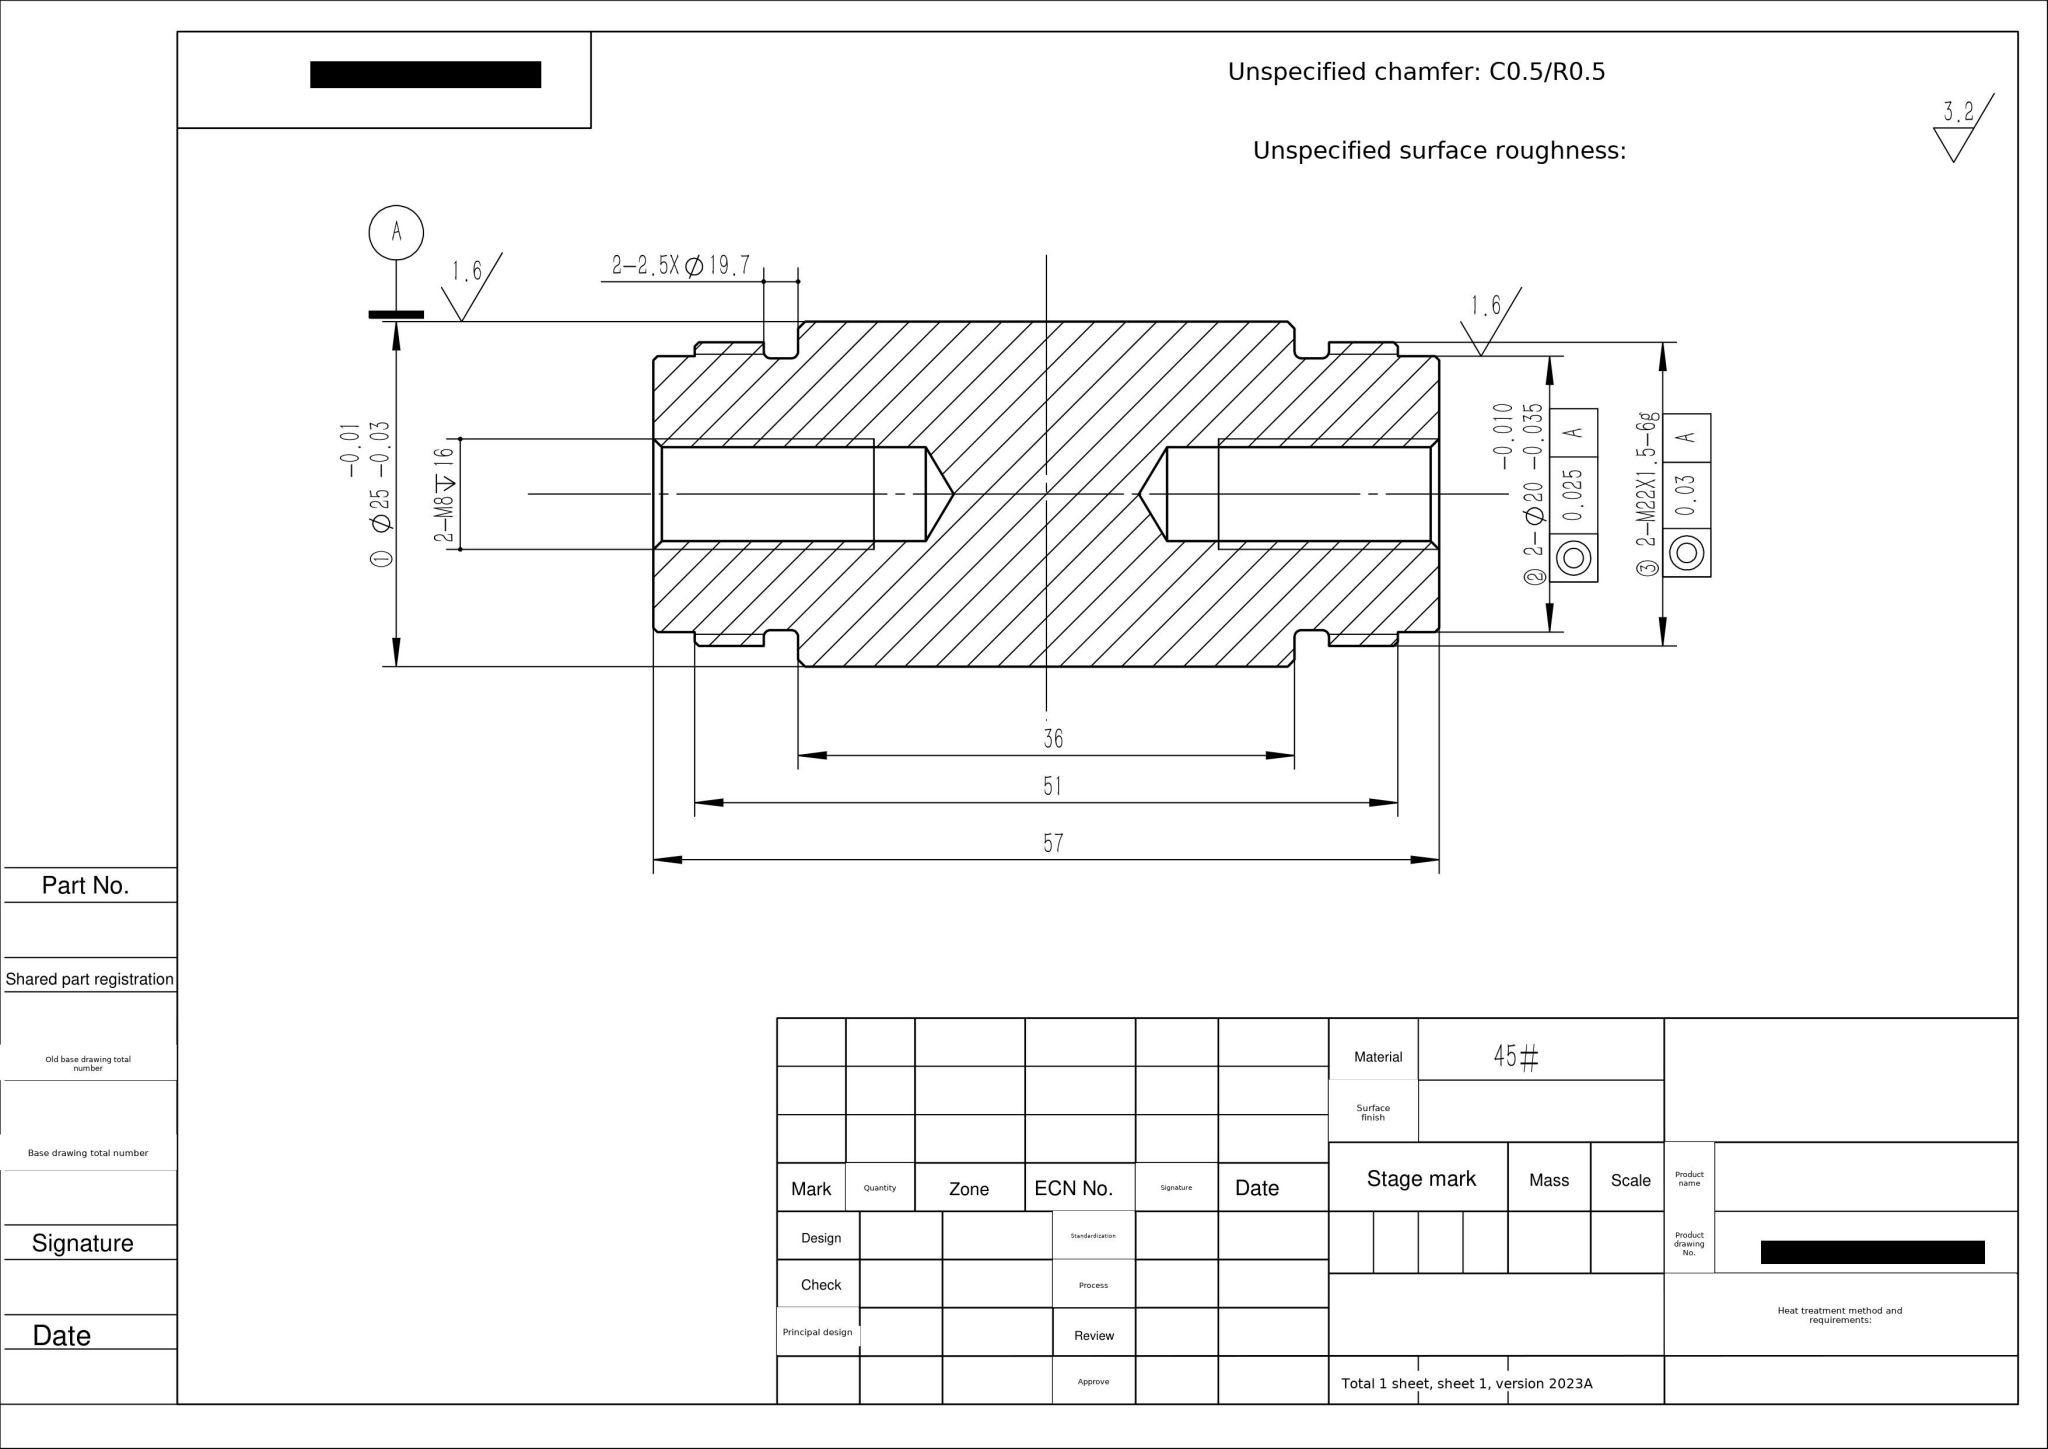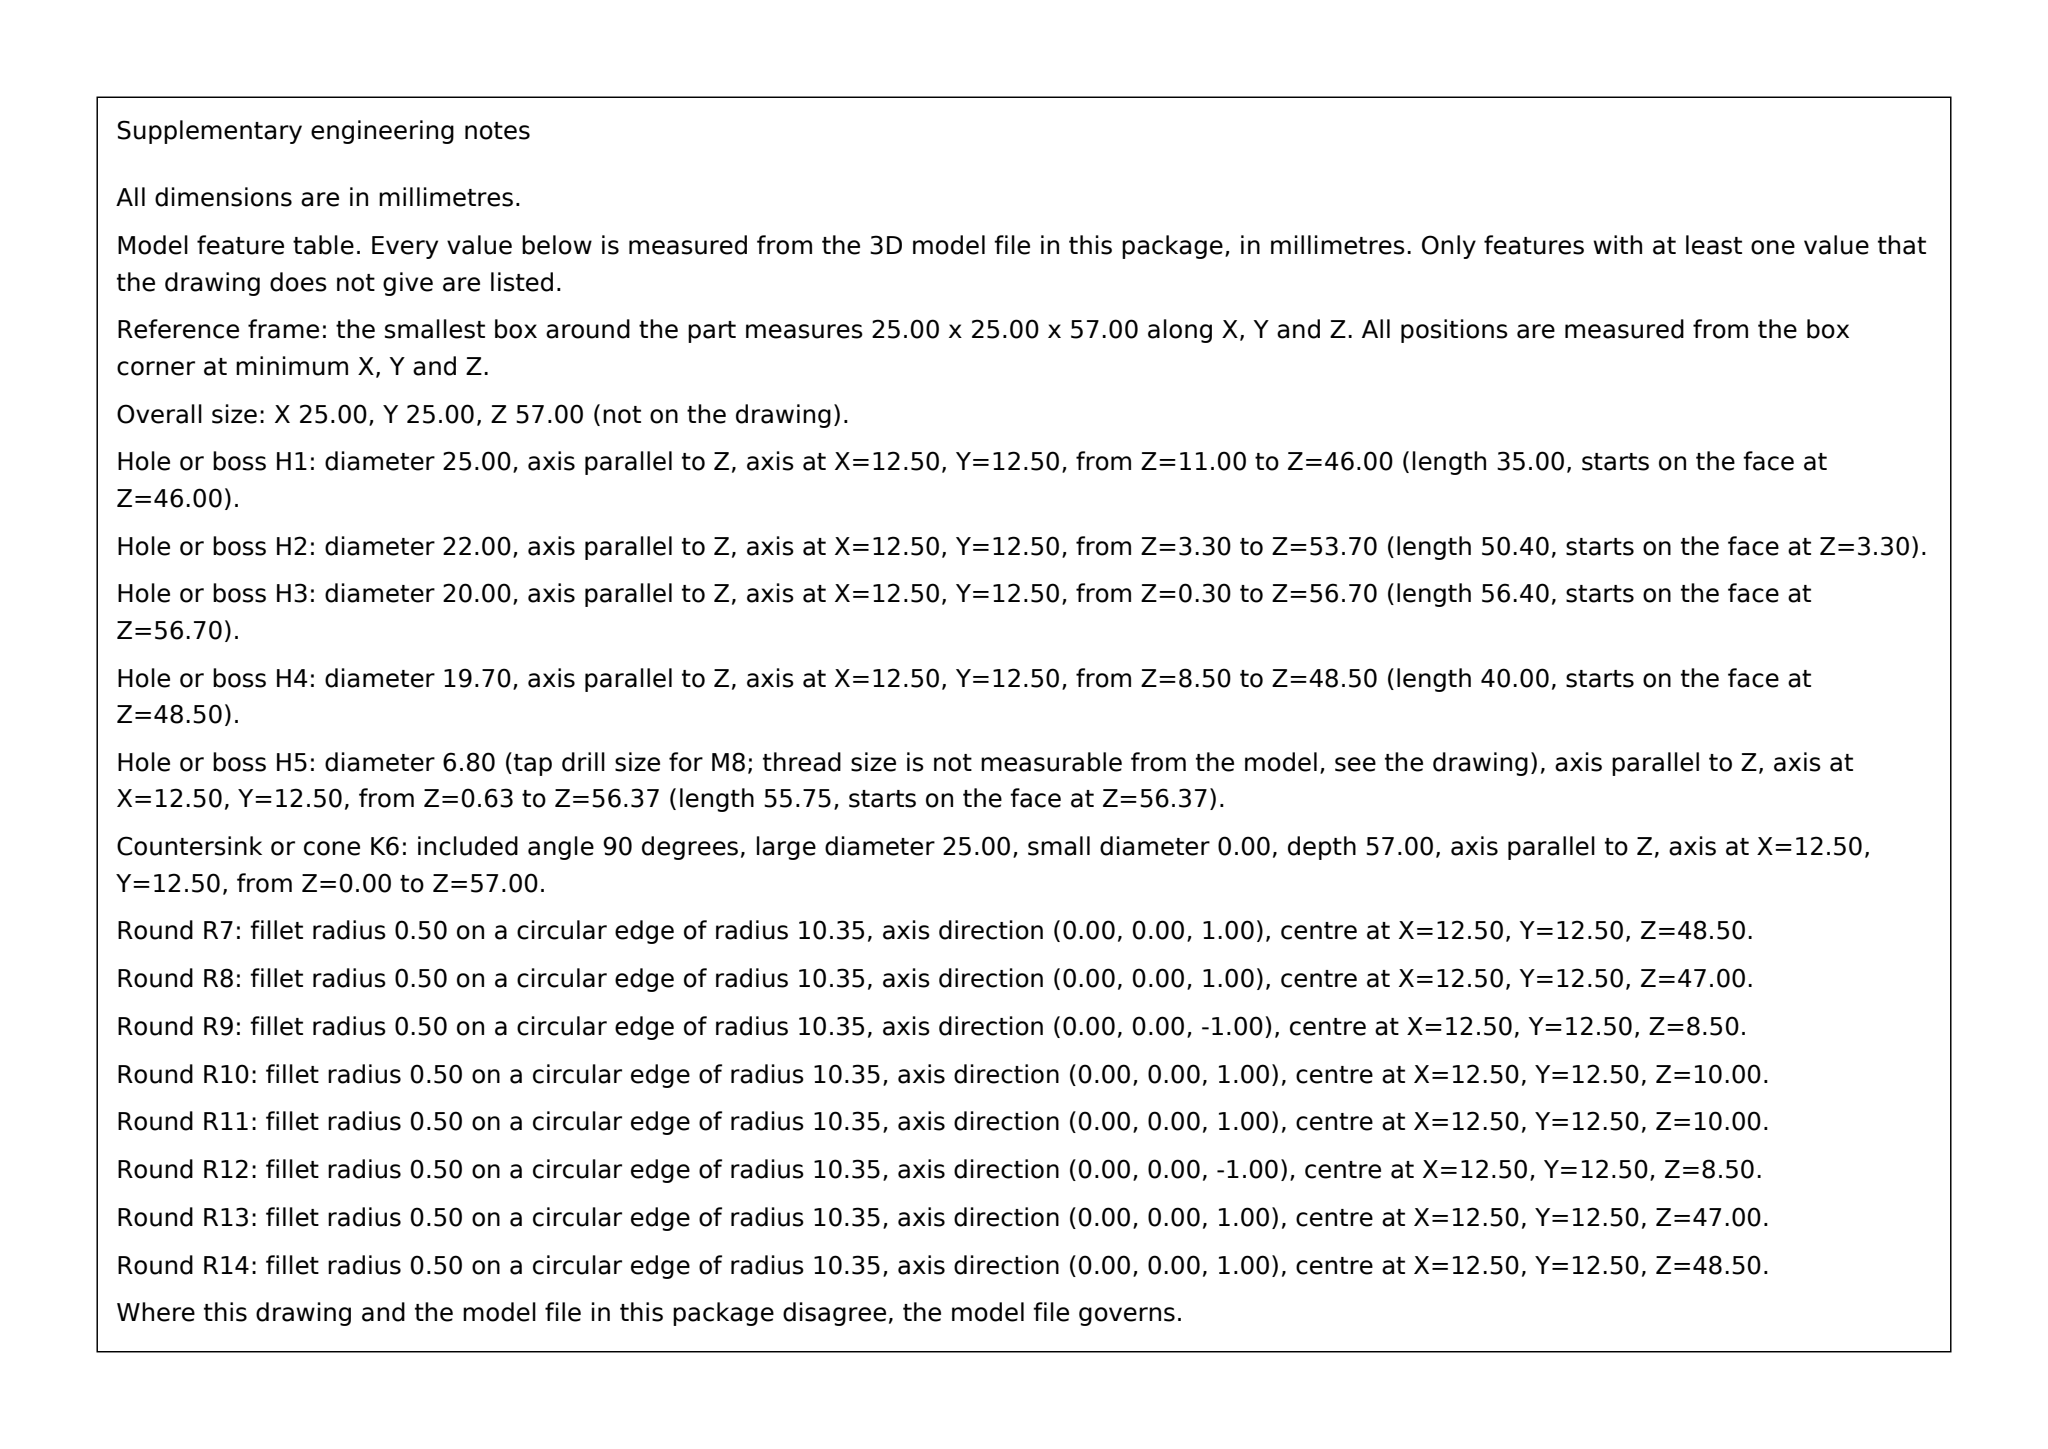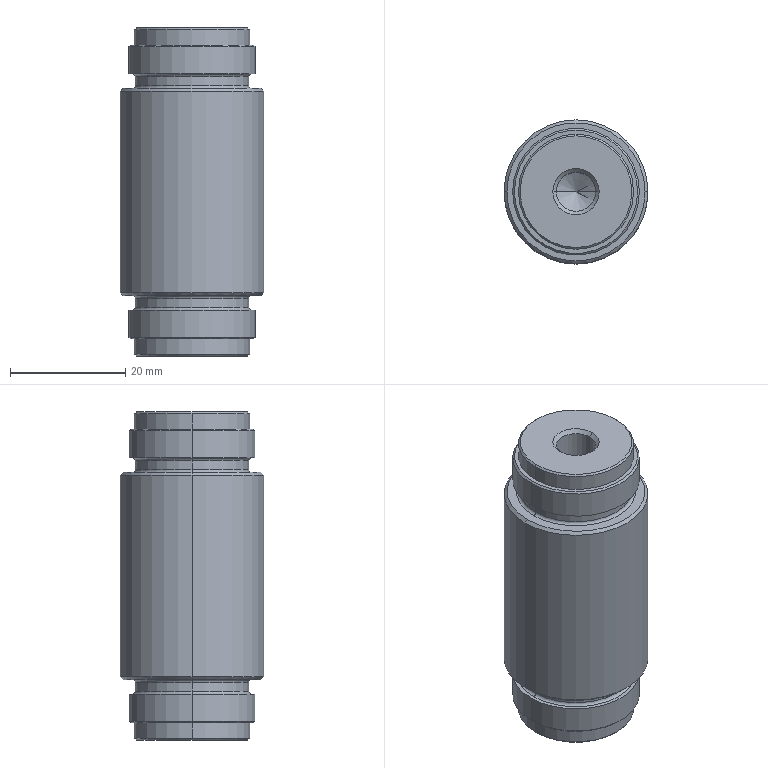Part | SolidWorks | mm | material 45# | 1 solid | 54 faces | box 25 x 25 x 57 mm | volume 23371 mm3 | cone 20 | cylinder 18 | torus 8 | plane 8 | commonest cylinder face diameters 22 x4 20 x4 6.8 x4 19.7 x4 25 x2
build123d program:
from build123d import *

# Parameters (mm, degrees)
SKETCH1_R                   = 12.5
BOSS_EXTRUDE1_DEPTH         = 18
CHAMFER1_SIZE               = 0.5
SKETCH2_R                   = 11
BOSS_EXTRUDE2_DEPTH         = 7.5
SKETCH3_R                   = 10
BOSS_EXTRUDE3_DEPTH         = 3
CHAMFER2_SIZE               = 0.3
M8_TAPPED_HOLE1_D           = 6.8
M8_TAPPED_HOLE1_DEPTH       = 19.75
M8_TAPPED_HOLE1_CSINK_D     = 8.05
M8_TAPPED_HOLE1_CSINK_ANGLE = 90
M8_TAPPED_HOLE1_TIP         = 2.043
M8_TAPPED_HOLE2_D           = 6.8
M8_TAPPED_HOLE2_DEPTH       = 19.75
M8_TAPPED_HOLE2_CSINK_D     = 8.05
M8_TAPPED_HOLE2_CSINK_ANGLE = 90
M8_TAPPED_HOLE2_TIP         = 2.043
SKETCH8_OUTSIDE_W           = 40.414
SKETCH8_OUTSIDE_H           = 40.414
SKETCH8_OUTSIDE_R           = 9.85
CUT_EXTRUDE1_DEPTH          = 2.5
FILLET1_R                   = 0.5


with BuildPart() as part:
    # Sketch1 → Boss-Extrude1 (new, symmetric)
    with BuildSketch(Plane.XY):
        Circle(SKETCH1_R)
    extrude(amount=BOSS_EXTRUDE1_DEPTH, both=True)

    # Chamfer1
    chamfer1_edges = [part.edges().sort_by_distance(p)[0] for p in [
        (-12.5, 0, -18),
        (-12.5, 0, 18),
    ]]
    chamfer(chamfer1_edges, length=CHAMFER1_SIZE)

    # Sketch2 → Boss-Extrude2 (add)
    with BuildSketch(Plane.XY.offset(18)):
        Circle(SKETCH2_R)
    boss_extrude2 = extrude(amount=BOSS_EXTRUDE2_DEPTH)

    # Mirror1: Boss-Extrude2 across plane
    add(boss_extrude2.mirror(Plane.XY))

    # Sketch3 → Boss-Extrude3 (add)
    with BuildSketch(Plane.XY.offset(25.5)):
        Circle(SKETCH3_R)
    boss_extrude3 = extrude(amount=BOSS_EXTRUDE3_DEPTH)

    # Mirror2: Boss-Extrude3 across plane
    add(boss_extrude3.mirror(Plane.XY))

    # Chamfer2
    chamfer2_edges = [part.edges().sort_by_distance(p)[0] for p in [
        (-11, 0, 25.5),
        (-11, 0, -25.5),
        (-10, 0, 28.5),
        (-10, 0, -28.5),
    ]]
    chamfer(chamfer2_edges, length=CHAMFER2_SIZE)

    # M8 Tapped Hole1
    with Locations(Plane.XY.offset(28.5)):
        with Locations((0, 0)):
            CounterSinkHole(M8_TAPPED_HOLE1_D / 2, M8_TAPPED_HOLE1_CSINK_D / 2, depth=M8_TAPPED_HOLE1_DEPTH, counter_sink_angle=M8_TAPPED_HOLE1_CSINK_ANGLE)
            with Locations((0, 0, -(M8_TAPPED_HOLE1_DEPTH + M8_TAPPED_HOLE1_TIP / 2))):  # 118° drill point
                Cone(0, M8_TAPPED_HOLE1_D / 2, M8_TAPPED_HOLE1_TIP, mode=Mode.SUBTRACT)

    # M8 Tapped Hole2
    with Locations(Plane(origin=(0, 0, -28.5), x_dir=(-1, 0, 0), z_dir=(0, 0, -1))):
        with Locations((0, 0)):
            CounterSinkHole(M8_TAPPED_HOLE2_D / 2, M8_TAPPED_HOLE2_CSINK_D / 2, depth=M8_TAPPED_HOLE2_DEPTH, counter_sink_angle=M8_TAPPED_HOLE2_CSINK_ANGLE)
            with Locations((0, 0, -(M8_TAPPED_HOLE2_DEPTH + M8_TAPPED_HOLE2_TIP / 2))):  # 118° drill point
                Cone(0, M8_TAPPED_HOLE2_D / 2, M8_TAPPED_HOLE2_TIP, mode=Mode.SUBTRACT)

    # Sketch8 outside → Cut-Extrude1 (cut)
    with BuildSketch(Plane.XY.offset(18)):
        Rectangle(SKETCH8_OUTSIDE_W, SKETCH8_OUTSIDE_H)
        Circle(SKETCH8_OUTSIDE_R, mode=Mode.SUBTRACT)
    cut_extrude1 = extrude(amount=CUT_EXTRUDE1_DEPTH, mode=Mode.SUBTRACT)

    # Mirror3: Cut-Extrude1 across plane
    add(cut_extrude1.mirror(Plane.XY), mode=Mode.SUBTRACT)

    # Fillet1
    fillet1_edges = [part.edges().sort_by_distance(p)[0] for p in [
        (-9.85, 0, 18),
        (-9.85, 0, 20.5),
        (-9.85, 0, -20.5),
        (-9.85, 0, -18),
    ]]
    fillet(fillet1_edges, radius=FILLET1_R)


solid = part.part